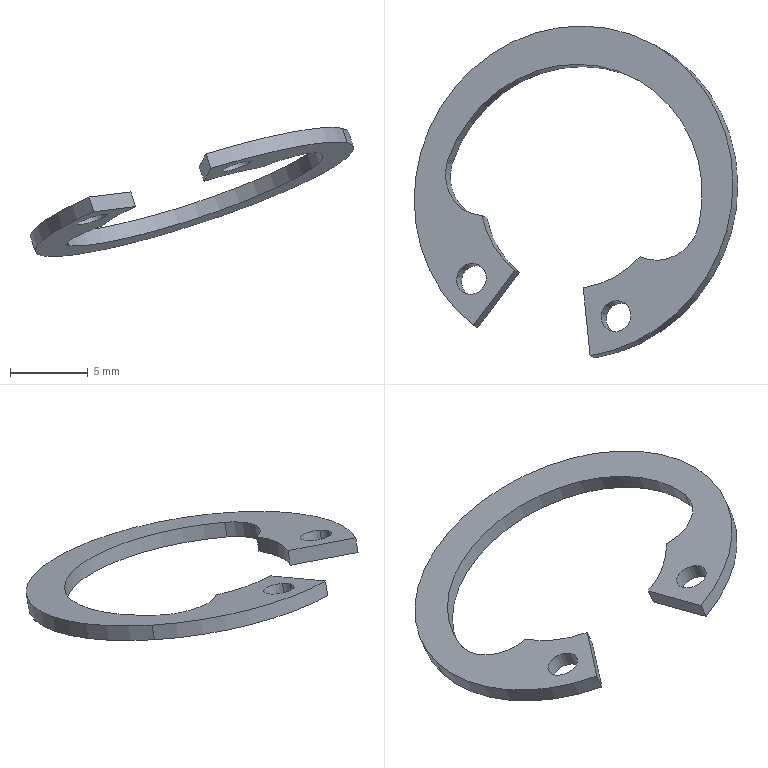Component | SolidWorks | FilmPressingSoilCoveringMechanism2Reverse-2_AttachedSoilDiskAssembly2-1_circlips for hole--type b gb-1 | 1 solid | 17 faces | box 20.75 x 21.29 x 8.29 mm | volume 139 mm3 | cylinder 13 | plane 4 | commonest cylinder face diameters 2 x4 5.6 x3 21.5 x3 12.6 x2 17.7 x1
build123d program:
from build123d import *

# Parameters (mm, degrees)
SKETCH1_R  = 1
BODY_DEPTH = 1


with BuildPart() as part:
    # Sketch1 → Body (new body)
    with BuildSketch(Plane.XY):
        with BuildLine():
            Line((-2.411, -5.82), (-4.114, -9.932))
            ThreePointArc((-4.114, -9.932), (0, 10.75), (4.114, -9.932))
            Line((4.114, -9.932), (2.411, -5.82))
            ThreePointArc((2.411, -5.82), (4.232, -4.667), (5.558, -2.966))
            ThreePointArc((5.558, -2.966), (7.908, -2.29), (8.831, -0.02556))
            ThreePointArc((8.831, -0.02556), (0, 8.25), (-8.831, -0.02556))
            ThreePointArc((-8.831, -0.02556), (-7.908, -2.29), (-5.558, -2.966))
            ThreePointArc((-5.558, -2.966), (-4.232, -4.667), (-2.411, -5.82))
        make_face()
        with Locations(Location((5.088, -7.057, 0), (0, 0, 180))):
            Circle(SKETCH1_R, mode=Mode.SUBTRACT)
        with Locations((-5.088, -7.057)):
            Circle(SKETCH1_R, mode=Mode.SUBTRACT)
    extrude(amount=-BODY_DEPTH)


solid = part.part

# Placed as in the assembly
solid = solid.moved(Location((-1925.591, -301.038, 2610.257), (-8.826, -18.019, -16.572)))
STEP:
#1=COLOUR_RGB('',0.7922,0.8196,0.9333);
#2=FILL_AREA_STYLE_COLOUR('',#1);
#3=FILL_AREA_STYLE('',(#2));
#4=SURFACE_STYLE_FILL_AREA(#3);
#5=SURFACE_SIDE_STYLE('',(#4));
#6=SURFACE_STYLE_USAGE(.BOTH.,#5);
#7=PRESENTATION_STYLE_ASSIGNMENT((#6));
#8=CARTESIAN_POINT('',(-76.033,-12.081,102.728));
#9=VERTEX_POINT('',#8);
#10=CARTESIAN_POINT('',(-76.104,-12.062,102.702));
#11=VERTEX_POINT('',#10);
#12=CARTESIAN_POINT('',(-76.069,-12.071,102.715));
#13=DIRECTION('',(0.3093,-0.1459,-0.9397));
#14=DIRECTION('',(0.9115,-0.2363,0.3367));
#15=AXIS2_PLACEMENT_3D('',#12,#13,#14);
#16=CIRCLE('',#15,0.03937);
#17=EDGE_CURVE('',#9,#11,#16,.T.);
#18=ORIENTED_EDGE('',*,*,#17,.F.);
#19=CARTESIAN_POINT('',(-76.021,-12.086,102.691));
#20=VERTEX_POINT('',#19);
#21=CARTESIAN_POINT('',(-76.033,-12.081,102.728));
#22=DIRECTION('',(0.3093,-0.1459,-0.9397));
#23=VECTOR('',#22,39.37);
#24=LINE('',#21,#23);
#25=EDGE_CURVE('',#9,#20,#24,.T.);
#26=ORIENTED_EDGE('',*,*,#25,.T.);
#27=CARTESIAN_POINT('',(-76.092,-12.068,102.665));
#28=VERTEX_POINT('',#27);
#29=CARTESIAN_POINT('',(-76.056,-12.077,102.678));
#30=DIRECTION('',(0.3093,-0.1459,-0.9397));
#31=DIRECTION('',(0.9115,-0.2363,0.3367));
#32=AXIS2_PLACEMENT_3D('',#29,#30,#31);
#33=CIRCLE('',#32,0.03937);
#34=EDGE_CURVE('',#20,#28,#33,.T.);
#35=ORIENTED_EDGE('',*,*,#34,.T.);
#36=CARTESIAN_POINT('',(-76.104,-12.062,102.702));
#37=DIRECTION('',(0.3093,-0.1459,-0.9397));
#38=VECTOR('',#37,39.37);
#39=LINE('',#36,#38);
#40=EDGE_CURVE('',#11,#28,#39,.T.);
#41=ORIENTED_EDGE('',*,*,#40,.F.);
#42=EDGE_LOOP('',(#18,#26,#35,#41));
#43=FACE_OUTER_BOUND('',#42,.T.);
#44=CARTESIAN_POINT('',(-76.069,-12.071,102.715));
#45=DIRECTION('',(0.3093,-0.1459,-0.9397));
#46=DIRECTION('',(-0.9115,0.2363,-0.3367));
#47=AXIS2_PLACEMENT_3D('',#44,#45,#46);
#48=CYLINDRICAL_SURFACE('',#47,0.03937);
#49=ADVANCED_FACE('',(#43),#48,.F.);
#50=CARTESIAN_POINT('',(-75.668,-12.175,102.863));
#51=VERTEX_POINT('',#50);
#52=CARTESIAN_POINT('',(-75.739,-12.157,102.837));
#53=VERTEX_POINT('',#52);
#54=CARTESIAN_POINT('',(-75.703,-12.166,102.85));
#55=DIRECTION('',(0.3093,-0.1459,-0.9397));
#56=DIRECTION('',(-0.9115,0.2363,-0.3367));
#57=AXIS2_PLACEMENT_3D('',#54,#55,#56);
#58=CIRCLE('',#57,0.03937);
#59=EDGE_CURVE('',#51,#53,#58,.T.);
#60=ORIENTED_EDGE('',*,*,#59,.F.);
#61=CARTESIAN_POINT('',(-75.655,-12.181,102.826));
#62=VERTEX_POINT('',#61);
#63=CARTESIAN_POINT('',(-75.668,-12.175,102.863));
#64=DIRECTION('',(0.3093,-0.1459,-0.9397));
#65=VECTOR('',#64,39.37);
#66=LINE('',#63,#65);
#67=EDGE_CURVE('',#51,#62,#66,.T.);
#68=ORIENTED_EDGE('',*,*,#67,.T.);
#69=CARTESIAN_POINT('',(-75.727,-12.163,102.8));
#70=VERTEX_POINT('',#69);
#71=CARTESIAN_POINT('',(-75.691,-12.172,102.813));
#72=DIRECTION('',(0.3093,-0.1459,-0.9397));
#73=DIRECTION('',(-0.9115,0.2363,-0.3367));
#74=AXIS2_PLACEMENT_3D('',#71,#72,#73);
#75=CIRCLE('',#74,0.03937);
#76=EDGE_CURVE('',#62,#70,#75,.T.);
#77=ORIENTED_EDGE('',*,*,#76,.T.);
#78=CARTESIAN_POINT('',(-75.739,-12.157,102.837));
#79=DIRECTION('',(0.3093,-0.1459,-0.9397));
#80=VECTOR('',#79,39.37);
#81=LINE('',#78,#80);
#82=EDGE_CURVE('',#53,#70,#81,.T.);
#83=ORIENTED_EDGE('',*,*,#82,.F.);
#84=EDGE_LOOP('',(#60,#68,#77,#83));
#85=FACE_OUTER_BOUND('',#84,.T.);
#86=CARTESIAN_POINT('',(-75.703,-12.166,102.85));
#87=DIRECTION('',(0.3093,-0.1459,-0.9397));
#88=DIRECTION('',(-0.9115,0.2363,-0.3367));
#89=AXIS2_PLACEMENT_3D('',#86,#87,#88);
#90=CYLINDRICAL_SURFACE('',#89,0.03937);
#91=ADVANCED_FACE('',(#85),#90,.F.);
#92=CARTESIAN_POINT('',(-76.128,-11.771,102.649));
#93=VERTEX_POINT('',#92);
#94=CARTESIAN_POINT('',(-76.13,-11.777,102.649));
#95=VERTEX_POINT('',#94);
#96=CARTESIAN_POINT('',(-76.03,-11.804,102.686));
#97=DIRECTION('',(-0.3093,0.1459,0.9397));
#98=DIRECTION('',(0.9115,-0.2363,0.3367));
#99=AXIS2_PLACEMENT_3D('',#96,#97,#98);
#100=CIRCLE('',#99,0.1102);
#101=EDGE_CURVE('',#93,#95,#100,.T.);
#102=ORIENTED_EDGE('',*,*,#101,.T.);
#103=CARTESIAN_POINT('',(-76.118,-11.783,102.612));
#104=VERTEX_POINT('',#103);
#105=CARTESIAN_POINT('',(-76.13,-11.777,102.649));
#106=DIRECTION('',(0.3093,-0.1459,-0.9397));
#107=VECTOR('',#106,39.37);
#108=LINE('',#105,#107);
#109=EDGE_CURVE('',#95,#104,#108,.T.);
#110=ORIENTED_EDGE('',*,*,#109,.T.);
#111=CARTESIAN_POINT('',(-76.116,-11.776,102.612));
#112=VERTEX_POINT('',#111);
#113=CARTESIAN_POINT('',(-76.017,-11.809,102.649));
#114=DIRECTION('',(-0.3093,0.1459,0.9397));
#115=DIRECTION('',(0.9115,-0.2363,0.3367));
#116=AXIS2_PLACEMENT_3D('',#113,#114,#115);
#117=CIRCLE('',#116,0.1102);
#118=EDGE_CURVE('',#112,#104,#117,.T.);
#119=ORIENTED_EDGE('',*,*,#118,.F.);
#120=CARTESIAN_POINT('',(-76.128,-11.771,102.649));
#121=DIRECTION('',(0.3093,-0.1459,-0.9397));
#122=VECTOR('',#121,39.37);
#123=LINE('',#120,#122);
#124=EDGE_CURVE('',#93,#112,#123,.T.);
#125=ORIENTED_EDGE('',*,*,#124,.F.);
#126=EDGE_LOOP('',(#102,#110,#119,#125));
#127=FACE_OUTER_BOUND('',#126,.T.);
#128=CARTESIAN_POINT('',(-76.03,-11.804,102.686));
#129=DIRECTION('',(0.3093,-0.1459,-0.9397));
#130=DIRECTION('',(-0.9115,0.2363,-0.3367));
#131=AXIS2_PLACEMENT_3D('',#128,#129,#130);
#132=CYLINDRICAL_SURFACE('',#131,0.1102);
#133=ADVANCED_FACE('',(#127),#132,.F.);
#134=CARTESIAN_POINT('',(-76.196,-11.752,102.624));
#135=VERTEX_POINT('',#134);
#136=CARTESIAN_POINT('',(-75.425,-11.952,102.909));
#137=VERTEX_POINT('',#136);
#138=CARTESIAN_POINT('',(-75.811,-11.852,102.766));
#139=DIRECTION('',(0.3093,-0.1459,-0.9397));
#140=DIRECTION('',(-0.9115,0.2363,-0.3367));
#141=AXIS2_PLACEMENT_3D('',#138,#139,#140);
#142=CIRCLE('',#141,0.4232);
#143=EDGE_CURVE('',#135,#137,#142,.T.);
#144=ORIENTED_EDGE('',*,*,#143,.T.);
#145=CARTESIAN_POINT('',(-75.413,-11.958,102.872));
#146=VERTEX_POINT('',#145);
#147=CARTESIAN_POINT('',(-75.425,-11.952,102.909));
#148=DIRECTION('',(0.3093,-0.1459,-0.9397));
#149=VECTOR('',#148,39.37);
#150=LINE('',#147,#149);
#151=EDGE_CURVE('',#137,#146,#150,.T.);
#152=ORIENTED_EDGE('',*,*,#151,.T.);
#153=CARTESIAN_POINT('',(-76.184,-11.758,102.587));
#154=VERTEX_POINT('',#153);
#155=CARTESIAN_POINT('',(-75.798,-11.858,102.729));
#156=DIRECTION('',(0.3093,-0.1459,-0.9397));
#157=DIRECTION('',(-0.9115,0.2363,-0.3367));
#158=AXIS2_PLACEMENT_3D('',#155,#156,#157);
#159=CIRCLE('',#158,0.4232);
#160=EDGE_CURVE('',#154,#146,#159,.T.);
#161=ORIENTED_EDGE('',*,*,#160,.F.);
#162=CARTESIAN_POINT('',(-76.196,-11.752,102.624));
#163=DIRECTION('',(0.3093,-0.1459,-0.9397));
#164=VECTOR('',#163,39.37);
#165=LINE('',#162,#164);
#166=EDGE_CURVE('',#135,#154,#165,.T.);
#167=ORIENTED_EDGE('',*,*,#166,.F.);
#168=EDGE_LOOP('',(#144,#152,#161,#167));
#169=FACE_OUTER_BOUND('',#168,.T.);
#170=CARTESIAN_POINT('',(-75.811,-11.852,102.766));
#171=DIRECTION('',(0.3093,-0.1459,-0.9397));
#172=DIRECTION('',(-0.9115,0.2363,-0.3367));
#173=AXIS2_PLACEMENT_3D('',#170,#171,#172);
#174=CYLINDRICAL_SURFACE('',#173,0.4232);
#175=ADVANCED_FACE('',(#169),#174,.T.);
#176=CARTESIAN_POINT('',(-76.064,-12.189,102.735));
#177=VERTEX_POINT('',#176);
#178=CARTESIAN_POINT('',(-75.811,-11.852,102.766));
#179=DIRECTION('',(0.3093,-0.1459,-0.9397));
#180=DIRECTION('',(-0.9115,0.2363,-0.3367));
#181=AXIS2_PLACEMENT_3D('',#178,#179,#180);
#182=CIRCLE('',#181,0.4232);
#183=EDGE_CURVE('',#177,#135,#182,.T.);
#184=ORIENTED_EDGE('',*,*,#183,.T.);
#185=ORIENTED_EDGE('',*,*,#166,.T.);
#186=CARTESIAN_POINT('',(-76.052,-12.195,102.698));
#187=VERTEX_POINT('',#186);
#188=CARTESIAN_POINT('',(-75.798,-11.858,102.729));
#189=DIRECTION('',(0.3093,-0.1459,-0.9397));
#190=DIRECTION('',(-0.9115,0.2363,-0.3367));
#191=AXIS2_PLACEMENT_3D('',#188,#189,#190);
#192=CIRCLE('',#191,0.4232);
#193=EDGE_CURVE('',#187,#154,#192,.T.);
#194=ORIENTED_EDGE('',*,*,#193,.F.);
#195=CARTESIAN_POINT('',(-76.064,-12.189,102.735));
#196=DIRECTION('',(0.3093,-0.1459,-0.9397));
#197=VECTOR('',#196,39.37);
#198=LINE('',#195,#197);
#199=EDGE_CURVE('',#177,#187,#198,.T.);
#200=ORIENTED_EDGE('',*,*,#199,.F.);
#201=EDGE_LOOP('',(#184,#185,#194,#200));
#202=FACE_OUTER_BOUND('',#201,.T.);
#203=CARTESIAN_POINT('',(-75.811,-11.852,102.766));
#204=DIRECTION('',(0.3093,-0.1459,-0.9397));
#205=DIRECTION('',(-0.9115,0.2363,-0.3367));
#206=AXIS2_PLACEMENT_3D('',#203,#204,#205);
#207=CYLINDRICAL_SURFACE('',#206,0.4232);
#208=ADVANCED_FACE('',(#202),#207,.T.);
#209=ORIENTED_EDGE('',*,*,#151,.F.);
#210=CARTESIAN_POINT('',(-75.769,-12.266,102.844));
#211=VERTEX_POINT('',#210);
#212=CARTESIAN_POINT('',(-75.811,-11.852,102.766));
#213=DIRECTION('',(0.3093,-0.1459,-0.9397));
#214=DIRECTION('',(-0.9115,0.2363,-0.3367));
#215=AXIS2_PLACEMENT_3D('',#212,#213,#214);
#216=CIRCLE('',#215,0.4232);
#217=EDGE_CURVE('',#137,#211,#216,.T.);
#218=ORIENTED_EDGE('',*,*,#217,.T.);
#219=CARTESIAN_POINT('',(-75.757,-12.272,102.807));
#220=VERTEX_POINT('',#219);
#221=CARTESIAN_POINT('',(-75.769,-12.266,102.844));
#222=DIRECTION('',(0.3093,-0.1459,-0.9397));
#223=VECTOR('',#222,39.37);
#224=LINE('',#221,#223);
#225=EDGE_CURVE('',#211,#220,#224,.T.);
#226=ORIENTED_EDGE('',*,*,#225,.T.);
#227=CARTESIAN_POINT('',(-75.798,-11.858,102.729));
#228=DIRECTION('',(0.3093,-0.1459,-0.9397));
#229=DIRECTION('',(-0.9115,0.2363,-0.3367));
#230=AXIS2_PLACEMENT_3D('',#227,#228,#229);
#231=CIRCLE('',#230,0.4232);
#232=EDGE_CURVE('',#146,#220,#231,.T.);
#233=ORIENTED_EDGE('',*,*,#232,.F.);
#234=EDGE_LOOP('',(#209,#218,#226,#233));
#235=FACE_OUTER_BOUND('',#234,.T.);
#236=CARTESIAN_POINT('',(-75.811,-11.852,102.766));
#237=DIRECTION('',(0.3093,-0.1459,-0.9397));
#238=DIRECTION('',(-0.9115,0.2363,-0.3367));
#239=AXIS2_PLACEMENT_3D('',#236,#237,#238);
#240=CYLINDRICAL_SURFACE('',#239,0.4232);
#241=ADVANCED_FACE('',(#235),#240,.T.);
#242=CARTESIAN_POINT('',(-75.947,-12.055,102.711));
#243=VERTEX_POINT('',#242);
#244=CARTESIAN_POINT('',(-75.947,-12.055,102.711));
#245=DIRECTION('',(-0.5994,-0.7971,-0.07355));
#246=VECTOR('',#245,39.37);
#247=LINE('',#244,#246);
#248=EDGE_CURVE('',#243,#187,#247,.T.);
#249=ORIENTED_EDGE('',*,*,#248,.F.);
#250=CARTESIAN_POINT('',(-75.959,-12.05,102.748));
#251=VERTEX_POINT('',#250);
#252=CARTESIAN_POINT('',(-75.959,-12.05,102.748));
#253=DIRECTION('',(0.3093,-0.1459,-0.9397));
#254=VECTOR('',#253,39.37);
#255=LINE('',#252,#254);
#256=EDGE_CURVE('',#251,#243,#255,.T.);
#257=ORIENTED_EDGE('',*,*,#256,.F.);
#258=CARTESIAN_POINT('',(-75.959,-12.05,102.748));
#259=DIRECTION('',(-0.5994,-0.7971,-0.07355));
#260=VECTOR('',#259,39.37);
#261=LINE('',#258,#260);
#262=EDGE_CURVE('',#251,#177,#261,.T.);
#263=ORIENTED_EDGE('',*,*,#262,.T.);
#264=ORIENTED_EDGE('',*,*,#199,.T.);
#265=EDGE_LOOP('',(#249,#257,#263,#264));
#266=FACE_OUTER_BOUND('',#265,.T.);
#267=CARTESIAN_POINT('',(-75.959,-12.05,102.748));
#268=DIRECTION('',(0.7383,-0.586,0.334));
#269=DIRECTION('',(-0.5994,-0.7971,-0.07355));
#270=AXIS2_PLACEMENT_3D('',#267,#268,#269);
#271=PLANE('',#270);
#272=ADVANCED_FACE('',(#266),#271,.T.);
#273=CARTESIAN_POINT('',(-76.03,-11.918,102.662));
#274=VERTEX_POINT('',#273);
#275=CARTESIAN_POINT('',(-75.798,-11.858,102.729));
#276=DIRECTION('',(-0.3093,0.1459,0.9397));
#277=DIRECTION('',(0.9115,-0.2363,0.3367));
#278=AXIS2_PLACEMENT_3D('',#275,#276,#277);
#279=CIRCLE('',#278,0.248);
#280=EDGE_CURVE('',#274,#243,#279,.T.);
#281=ORIENTED_EDGE('',*,*,#280,.F.);
#282=CARTESIAN_POINT('',(-76.042,-11.912,102.699));
#283=VERTEX_POINT('',#282);
#284=CARTESIAN_POINT('',(-76.042,-11.912,102.699));
#285=DIRECTION('',(0.3093,-0.1459,-0.9397));
#286=VECTOR('',#285,39.37);
#287=LINE('',#284,#286);
#288=EDGE_CURVE('',#283,#274,#287,.T.);
#289=ORIENTED_EDGE('',*,*,#288,.F.);
#290=CARTESIAN_POINT('',(-75.811,-11.852,102.766));
#291=DIRECTION('',(-0.3093,0.1459,0.9397));
#292=DIRECTION('',(0.9115,-0.2363,0.3367));
#293=AXIS2_PLACEMENT_3D('',#290,#291,#292);
#294=CIRCLE('',#293,0.248);
#295=EDGE_CURVE('',#283,#251,#294,.T.);
#296=ORIENTED_EDGE('',*,*,#295,.T.);
#297=ORIENTED_EDGE('',*,*,#256,.T.);
#298=EDGE_LOOP('',(#281,#289,#296,#297));
#299=FACE_OUTER_BOUND('',#298,.T.);
#300=CARTESIAN_POINT('',(-75.811,-11.852,102.766));
#301=DIRECTION('',(0.3093,-0.1459,-0.9397));
#302=DIRECTION('',(-0.9115,0.2363,-0.3367));
#303=AXIS2_PLACEMENT_3D('',#300,#301,#302);
#304=CYLINDRICAL_SURFACE('',#303,0.248);
#305=ADVANCED_FACE('',(#299),#304,.F.);
#306=ORIENTED_EDGE('',*,*,#109,.F.);
#307=CARTESIAN_POINT('',(-76.03,-11.804,102.686));
#308=DIRECTION('',(-0.3093,0.1459,0.9397));
#309=DIRECTION('',(0.9115,-0.2363,0.3367));
#310=AXIS2_PLACEMENT_3D('',#307,#308,#309);
#311=CIRCLE('',#310,0.1102);
#312=EDGE_CURVE('',#95,#283,#311,.T.);
#313=ORIENTED_EDGE('',*,*,#312,.T.);
#314=ORIENTED_EDGE('',*,*,#288,.T.);
#315=CARTESIAN_POINT('',(-76.017,-11.809,102.649));
#316=DIRECTION('',(-0.3093,0.1459,0.9397));
#317=DIRECTION('',(0.9115,-0.2363,0.3367));
#318=AXIS2_PLACEMENT_3D('',#315,#316,#317);
#319=CIRCLE('',#318,0.1102);
#320=EDGE_CURVE('',#104,#274,#319,.T.);
#321=ORIENTED_EDGE('',*,*,#320,.F.);
#322=EDGE_LOOP('',(#306,#313,#314,#321));
#323=FACE_OUTER_BOUND('',#322,.T.);
#324=CARTESIAN_POINT('',(-76.03,-11.804,102.686));
#325=DIRECTION('',(0.3093,-0.1459,-0.9397));
#326=DIRECTION('',(-0.9115,0.2363,-0.3367));
#327=AXIS2_PLACEMENT_3D('',#324,#325,#326);
#328=CYLINDRICAL_SURFACE('',#327,0.1102);
#329=ADVANCED_FACE('',(#323),#328,.F.);
#330=CARTESIAN_POINT('',(-75.482,-11.941,102.846));
#331=VERTEX_POINT('',#330);
#332=CARTESIAN_POINT('',(-75.805,-11.88,102.73));
#333=DIRECTION('',(-0.3093,0.1459,0.9397));
#334=DIRECTION('',(-0.9115,0.2363,-0.3367));
#335=AXIS2_PLACEMENT_3D('',#332,#333,#334);
#336=CIRCLE('',#335,0.3484);
#337=EDGE_CURVE('',#331,#112,#336,.T.);
#338=ORIENTED_EDGE('',*,*,#337,.F.);
#339=CARTESIAN_POINT('',(-75.494,-11.935,102.883));
#340=VERTEX_POINT('',#339);
#341=CARTESIAN_POINT('',(-75.494,-11.935,102.883));
#342=DIRECTION('',(0.3093,-0.1459,-0.9397));
#343=VECTOR('',#342,39.37);
#344=LINE('',#341,#343);
#345=EDGE_CURVE('',#340,#331,#344,.T.);
#346=ORIENTED_EDGE('',*,*,#345,.F.);
#347=CARTESIAN_POINT('',(-75.817,-11.875,102.767));
#348=DIRECTION('',(-0.3093,0.1459,0.9397));
#349=DIRECTION('',(-0.9115,0.2363,-0.3367));
#350=AXIS2_PLACEMENT_3D('',#347,#348,#349);
#351=CIRCLE('',#350,0.3484);
#352=EDGE_CURVE('',#340,#93,#351,.T.);
#353=ORIENTED_EDGE('',*,*,#352,.T.);
#354=ORIENTED_EDGE('',*,*,#124,.T.);
#355=EDGE_LOOP('',(#338,#346,#353,#354));
#356=FACE_OUTER_BOUND('',#355,.T.);
#357=CARTESIAN_POINT('',(-75.817,-11.875,102.767));
#358=DIRECTION('',(0.3093,-0.1459,-0.9397));
#359=DIRECTION('',(-0.9115,0.2363,-0.3367));
#360=AXIS2_PLACEMENT_3D('',#357,#358,#359);
#361=CYLINDRICAL_SURFACE('',#360,0.3484);
#362=ADVANCED_FACE('',(#356),#361,.F.);
#363=CARTESIAN_POINT('',(-75.631,-12.022,102.81));
#364=VERTEX_POINT('',#363);
#365=CARTESIAN_POINT('',(-75.584,-11.922,102.81));
#366=DIRECTION('',(-0.3093,0.1459,0.9397));
#367=DIRECTION('',(-0.9115,0.2363,-0.3367));
#368=AXIS2_PLACEMENT_3D('',#365,#366,#367);
#369=CIRCLE('',#368,0.1102);
#370=EDGE_CURVE('',#364,#331,#369,.T.);
#371=ORIENTED_EDGE('',*,*,#370,.F.);
#372=CARTESIAN_POINT('',(-75.643,-12.016,102.847));
#373=VERTEX_POINT('',#372);
#374=CARTESIAN_POINT('',(-75.643,-12.016,102.847));
#375=DIRECTION('',(0.3093,-0.1459,-0.9397));
#376=VECTOR('',#375,39.37);
#377=LINE('',#374,#376);
#378=EDGE_CURVE('',#373,#364,#377,.T.);
#379=ORIENTED_EDGE('',*,*,#378,.F.);
#380=CARTESIAN_POINT('',(-75.596,-11.916,102.847));
#381=DIRECTION('',(-0.3093,0.1459,0.9397));
#382=DIRECTION('',(-0.9115,0.2363,-0.3367));
#383=AXIS2_PLACEMENT_3D('',#380,#381,#382);
#384=CIRCLE('',#383,0.1102);
#385=EDGE_CURVE('',#373,#340,#384,.T.);
#386=ORIENTED_EDGE('',*,*,#385,.T.);
#387=ORIENTED_EDGE('',*,*,#345,.T.);
#388=EDGE_LOOP('',(#371,#379,#386,#387));
#389=FACE_OUTER_BOUND('',#388,.T.);
#390=CARTESIAN_POINT('',(-75.596,-11.916,102.847));
#391=DIRECTION('',(0.3093,-0.1459,-0.9397));
#392=DIRECTION('',(-0.9115,0.2363,-0.3367));
#393=AXIS2_PLACEMENT_3D('',#390,#391,#392);
#394=CYLINDRICAL_SURFACE('',#393,0.1102);
#395=ADVANCED_FACE('',(#389),#394,.F.);
#396=CARTESIAN_POINT('',(-75.774,-12.1,102.775));
#397=VERTEX_POINT('',#396);
#398=CARTESIAN_POINT('',(-75.798,-11.858,102.729));
#399=DIRECTION('',(-0.3093,0.1459,0.9397));
#400=DIRECTION('',(-0.9115,0.2363,-0.3367));
#401=AXIS2_PLACEMENT_3D('',#398,#399,#400);
#402=CIRCLE('',#401,0.248);
#403=EDGE_CURVE('',#397,#364,#402,.T.);
#404=ORIENTED_EDGE('',*,*,#403,.F.);
#405=CARTESIAN_POINT('',(-75.786,-12.094,102.812));
#406=VERTEX_POINT('',#405);
#407=CARTESIAN_POINT('',(-75.786,-12.094,102.812));
#408=DIRECTION('',(0.3093,-0.1459,-0.9397));
#409=VECTOR('',#408,39.37);
#410=LINE('',#407,#409);
#411=EDGE_CURVE('',#406,#397,#410,.T.);
#412=ORIENTED_EDGE('',*,*,#411,.F.);
#413=CARTESIAN_POINT('',(-75.811,-11.852,102.766));
#414=DIRECTION('',(-0.3093,0.1459,0.9397));
#415=DIRECTION('',(-0.9115,0.2363,-0.3367));
#416=AXIS2_PLACEMENT_3D('',#413,#414,#415);
#417=CIRCLE('',#416,0.248);
#418=EDGE_CURVE('',#406,#373,#417,.T.);
#419=ORIENTED_EDGE('',*,*,#418,.T.);
#420=ORIENTED_EDGE('',*,*,#378,.T.);
#421=EDGE_LOOP('',(#404,#412,#419,#420));
#422=FACE_OUTER_BOUND('',#421,.T.);
#423=CARTESIAN_POINT('',(-75.811,-11.852,102.766));
#424=DIRECTION('',(0.3093,-0.1459,-0.9397));
#425=DIRECTION('',(-0.9115,0.2363,-0.3367));
#426=AXIS2_PLACEMENT_3D('',#423,#424,#425);
#427=CYLINDRICAL_SURFACE('',#426,0.248);
#428=ADVANCED_FACE('',(#422),#427,.F.);
#429=CARTESIAN_POINT('',(-75.774,-12.1,102.775));
#430=DIRECTION('',(-0.09822,0.978,-0.1842));
#431=VECTOR('',#430,39.37);
#432=LINE('',#429,#431);
#433=EDGE_CURVE('',#220,#397,#432,.T.);
#434=ORIENTED_EDGE('',*,*,#433,.F.);
#435=ORIENTED_EDGE('',*,*,#225,.F.);
#436=CARTESIAN_POINT('',(-75.786,-12.094,102.812));
#437=DIRECTION('',(-0.09822,0.978,-0.1842));
#438=VECTOR('',#437,39.37);
#439=LINE('',#436,#438);
#440=EDGE_CURVE('',#211,#406,#439,.T.);
#441=ORIENTED_EDGE('',*,*,#440,.T.);
#442=ORIENTED_EDGE('',*,*,#411,.T.);
#443=EDGE_LOOP('',(#434,#435,#441,#442));
#444=FACE_OUTER_BOUND('',#443,.T.);
#445=CARTESIAN_POINT('',(-75.786,-12.094,102.812));
#446=DIRECTION('',(-0.9459,-0.1493,-0.2882));
#447=DIRECTION('',(-0.09822,0.978,-0.1842));
#448=AXIS2_PLACEMENT_3D('',#445,#446,#447);
#449=PLANE('',#448);
#450=ADVANCED_FACE('',(#444),#449,.T.);
#451=CARTESIAN_POINT('',(-76.069,-12.071,102.715));
#452=DIRECTION('',(0.3093,-0.1459,-0.9397));
#453=DIRECTION('',(0.9115,-0.2363,0.3367));
#454=AXIS2_PLACEMENT_3D('',#451,#452,#453);
#455=CIRCLE('',#454,0.03937);
#456=EDGE_CURVE('',#11,#9,#455,.T.);
#457=ORIENTED_EDGE('',*,*,#456,.T.);
#458=ORIENTED_EDGE('',*,*,#17,.T.);
#459=EDGE_LOOP('',(#457,#458));
#460=FACE_BOUND('',#459,.T.);
#461=CARTESIAN_POINT('',(-75.703,-12.166,102.85));
#462=DIRECTION('',(0.3093,-0.1459,-0.9397));
#463=DIRECTION('',(-0.9115,0.2363,-0.3367));
#464=AXIS2_PLACEMENT_3D('',#461,#462,#463);
#465=CIRCLE('',#464,0.03937);
#466=EDGE_CURVE('',#53,#51,#465,.T.);
#467=ORIENTED_EDGE('',*,*,#466,.T.);
#468=ORIENTED_EDGE('',*,*,#59,.T.);
#469=EDGE_LOOP('',(#467,#468));
#470=FACE_BOUND('',#469,.T.);
#471=ORIENTED_EDGE('',*,*,#183,.F.);
#472=ORIENTED_EDGE('',*,*,#262,.F.);
#473=ORIENTED_EDGE('',*,*,#295,.F.);
#474=ORIENTED_EDGE('',*,*,#312,.F.);
#475=ORIENTED_EDGE('',*,*,#101,.F.);
#476=ORIENTED_EDGE('',*,*,#352,.F.);
#477=ORIENTED_EDGE('',*,*,#385,.F.);
#478=ORIENTED_EDGE('',*,*,#418,.F.);
#479=ORIENTED_EDGE('',*,*,#440,.F.);
#480=ORIENTED_EDGE('',*,*,#217,.F.);
#481=ORIENTED_EDGE('',*,*,#143,.F.);
#482=EDGE_LOOP('',(#471,#472,#473,#474,#475,#476,#477,#478,#479,#480,#481));
#483=FACE_OUTER_BOUND('',#482,.T.);
#484=CARTESIAN_POINT('',(-75.811,-11.852,102.766));
#485=DIRECTION('',(0.3093,-0.1459,-0.9397));
#486=DIRECTION('',(-0.9115,0.2363,-0.3367));
#487=AXIS2_PLACEMENT_3D('',#484,#485,#486);
#488=PLANE('',#487);
#489=ADVANCED_FACE('',(#460,#470,#483),#488,.F.);
#490=CARTESIAN_POINT('',(-76.056,-12.077,102.678));
#491=DIRECTION('',(0.3093,-0.1459,-0.9397));
#492=DIRECTION('',(0.9115,-0.2363,0.3367));
#493=AXIS2_PLACEMENT_3D('',#490,#491,#492);
#494=CIRCLE('',#493,0.03937);
#495=EDGE_CURVE('',#28,#20,#494,.T.);
#496=ORIENTED_EDGE('',*,*,#495,.F.);
#497=ORIENTED_EDGE('',*,*,#34,.F.);
#498=EDGE_LOOP('',(#496,#497));
#499=FACE_BOUND('',#498,.T.);
#500=CARTESIAN_POINT('',(-75.691,-12.172,102.813));
#501=DIRECTION('',(0.3093,-0.1459,-0.9397));
#502=DIRECTION('',(-0.9115,0.2363,-0.3367));
#503=AXIS2_PLACEMENT_3D('',#500,#501,#502);
#504=CIRCLE('',#503,0.03937);
#505=EDGE_CURVE('',#70,#62,#504,.T.);
#506=ORIENTED_EDGE('',*,*,#505,.F.);
#507=ORIENTED_EDGE('',*,*,#76,.F.);
#508=EDGE_LOOP('',(#506,#507));
#509=FACE_BOUND('',#508,.T.);
#510=ORIENTED_EDGE('',*,*,#193,.T.);
#511=ORIENTED_EDGE('',*,*,#160,.T.);
#512=ORIENTED_EDGE('',*,*,#232,.T.);
#513=ORIENTED_EDGE('',*,*,#433,.T.);
#514=ORIENTED_EDGE('',*,*,#403,.T.);
#515=ORIENTED_EDGE('',*,*,#370,.T.);
#516=ORIENTED_EDGE('',*,*,#337,.T.);
#517=ORIENTED_EDGE('',*,*,#118,.T.);
#518=ORIENTED_EDGE('',*,*,#320,.T.);
#519=ORIENTED_EDGE('',*,*,#280,.T.);
#520=ORIENTED_EDGE('',*,*,#248,.T.);
#521=EDGE_LOOP('',(#510,#511,#512,#513,#514,#515,#516,#517,#518,#519,#520));
#522=FACE_OUTER_BOUND('',#521,.T.);
#523=CARTESIAN_POINT('',(-75.798,-11.858,102.729));
#524=DIRECTION('',(0.3093,-0.1459,-0.9397));
#525=DIRECTION('',(-0.9115,0.2363,-0.3367));
#526=AXIS2_PLACEMENT_3D('',#523,#524,#525);
#527=PLANE('',#526);
#528=ADVANCED_FACE('',(#499,#509,#522),#527,.T.);
#529=ORIENTED_EDGE('',*,*,#67,.F.);
#530=ORIENTED_EDGE('',*,*,#466,.F.);
#531=ORIENTED_EDGE('',*,*,#82,.T.);
#532=ORIENTED_EDGE('',*,*,#505,.T.);
#533=EDGE_LOOP('',(#529,#530,#531,#532));
#534=FACE_OUTER_BOUND('',#533,.T.);
#535=CARTESIAN_POINT('',(-75.703,-12.166,102.85));
#536=DIRECTION('',(0.3093,-0.1459,-0.9397));
#537=DIRECTION('',(-0.9115,0.2363,-0.3367));
#538=AXIS2_PLACEMENT_3D('',#535,#536,#537);
#539=CYLINDRICAL_SURFACE('',#538,0.03937);
#540=ADVANCED_FACE('',(#534),#539,.F.);
#541=ORIENTED_EDGE('',*,*,#25,.F.);
#542=ORIENTED_EDGE('',*,*,#456,.F.);
#543=ORIENTED_EDGE('',*,*,#40,.T.);
#544=ORIENTED_EDGE('',*,*,#495,.T.);
#545=EDGE_LOOP('',(#541,#542,#543,#544));
#546=FACE_OUTER_BOUND('',#545,.T.);
#547=CARTESIAN_POINT('',(-76.069,-12.071,102.715));
#548=DIRECTION('',(0.3093,-0.1459,-0.9397));
#549=DIRECTION('',(-0.9115,0.2363,-0.3367));
#550=AXIS2_PLACEMENT_3D('',#547,#548,#549);
#551=CYLINDRICAL_SURFACE('',#550,0.03937);
#552=ADVANCED_FACE('',(#546),#551,.F.);
#553=CLOSED_SHELL('',(#49,#91,#133,#175,#208,#241,#272,#305,#329,#362,#395,#428,#450,#489,#528,#540,#552));
#554=MANIFOLD_SOLID_BREP('',#553);
#555=STYLED_ITEM('',(#7),#554);
#556=PRESENTATION_LAYER_ASSIGNMENT('','',(#555));
#557=(LENGTH_UNIT()NAMED_UNIT(*)SI_UNIT($,.METRE.));
#558=LENGTH_MEASURE_WITH_UNIT(LENGTH_MEASURE(0.0254),#557);
#559=DIMENSIONAL_EXPONENTS(1.,0.,0.,0.,0.,0.,0.);
#560=(CONVERSION_BASED_UNIT('',#558)LENGTH_UNIT()NAMED_UNIT(#559));
#561=UNCERTAINTY_MEASURE_WITH_UNIT(LENGTH_MEASURE(0.00001),#560,'','');
#562=(NAMED_UNIT(*)PLANE_ANGLE_UNIT()SI_UNIT($,.RADIAN.));
#563=(NAMED_UNIT(*)SI_UNIT($,.STERADIAN.)SOLID_ANGLE_UNIT());
#564=(GEOMETRIC_REPRESENTATION_CONTEXT(3)GLOBAL_UNCERTAINTY_ASSIGNED_CONTEXT((#561))GLOBAL_UNIT_ASSIGNED_CONTEXT((#560,#562,#563))REPRESENTATION_CONTEXT('',''));
#565=MECHANICAL_DESIGN_GEOMETRIC_PRESENTATION_REPRESENTATION('',(#555),#564);
#566=CARTESIAN_POINT('',(0.,0.,0.));
#567=DIRECTION('',(0.,0.,1.));
#568=DIRECTION('',(1.,0.,0.));
#569=AXIS2_PLACEMENT_3D('',#566,#567,#568);
#570=(LENGTH_UNIT()NAMED_UNIT(*)SI_UNIT($,.METRE.));
#571=LENGTH_MEASURE_WITH_UNIT(LENGTH_MEASURE(0.0254),#570);
#572=DIMENSIONAL_EXPONENTS(1.,0.,0.,0.,0.,0.,0.);
#573=(CONVERSION_BASED_UNIT('',#571)LENGTH_UNIT()NAMED_UNIT(#572));
#574=UNCERTAINTY_MEASURE_WITH_UNIT(LENGTH_MEASURE(0.00001),#573,'','');
#575=(NAMED_UNIT(*)PLANE_ANGLE_UNIT()SI_UNIT($,.RADIAN.));
#576=(NAMED_UNIT(*)SI_UNIT($,.STERADIAN.)SOLID_ANGLE_UNIT());
#577=(GEOMETRIC_REPRESENTATION_CONTEXT(3)GLOBAL_UNCERTAINTY_ASSIGNED_CONTEXT((#574))GLOBAL_UNIT_ASSIGNED_CONTEXT((#573,#575,#576))REPRESENTATION_CONTEXT('',''));
#578=ADVANCED_BREP_SHAPE_REPRESENTATION('',(#554,#569),#577);